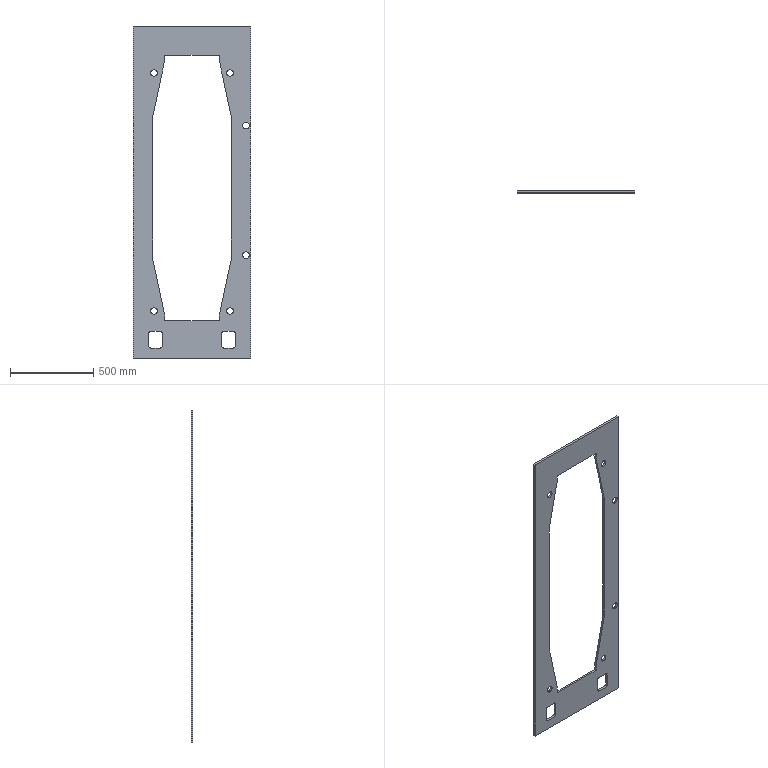Component | NX | CH3404_5-7 | 1 solid | 40 faces | volume 8407582 mm3 | plane 26 | cylinder 14 | commonest cylinder face diameters 20 x8 40 x6